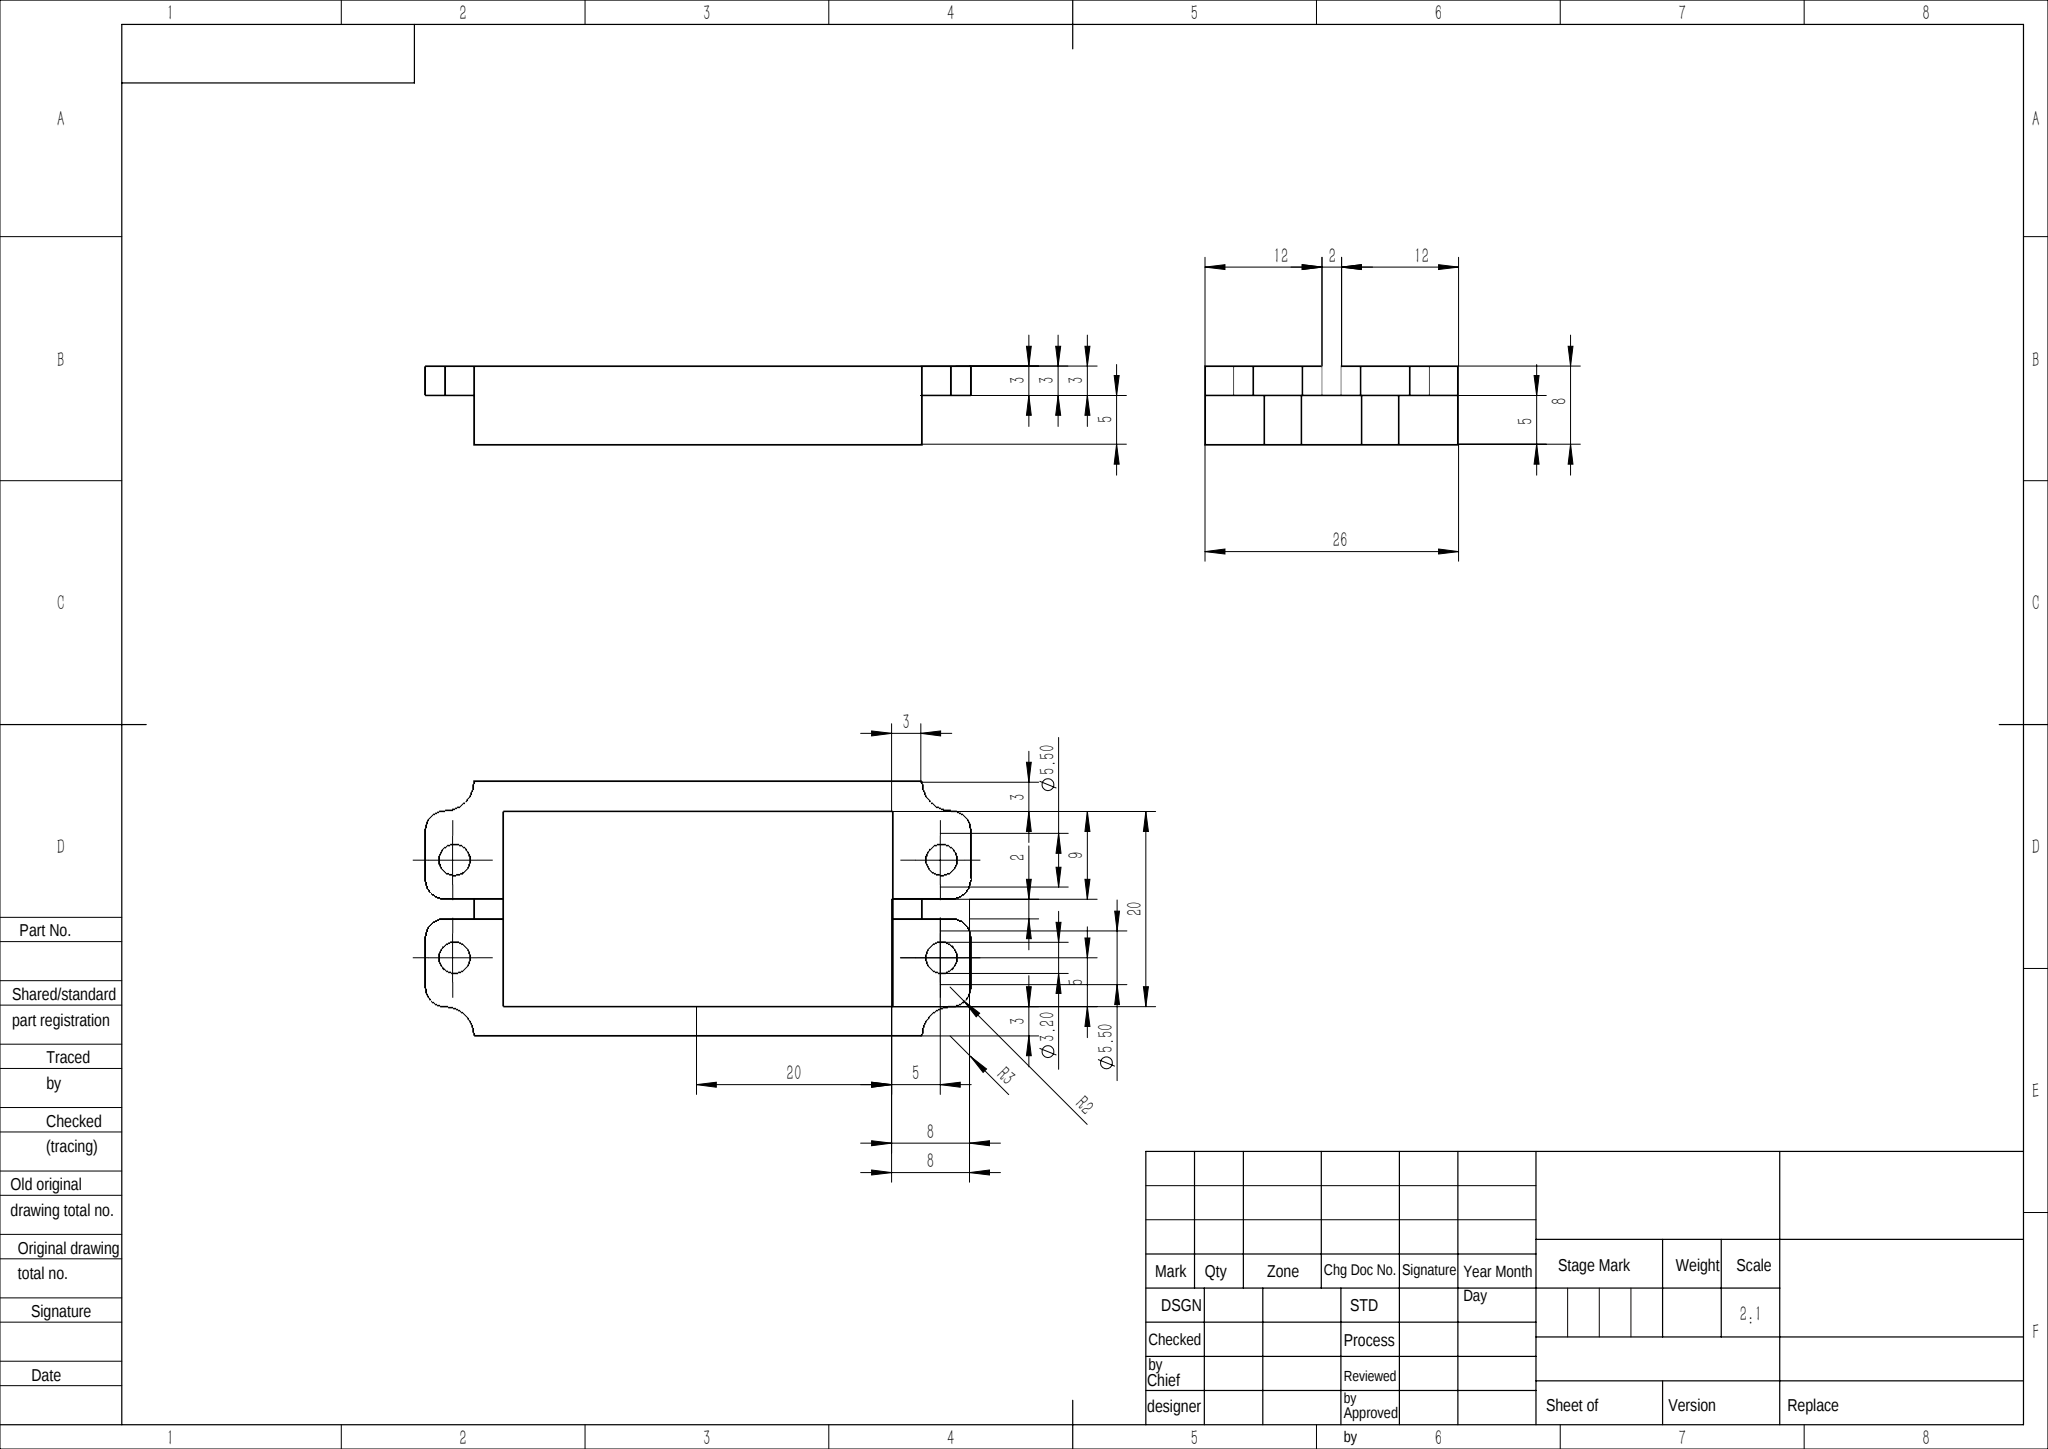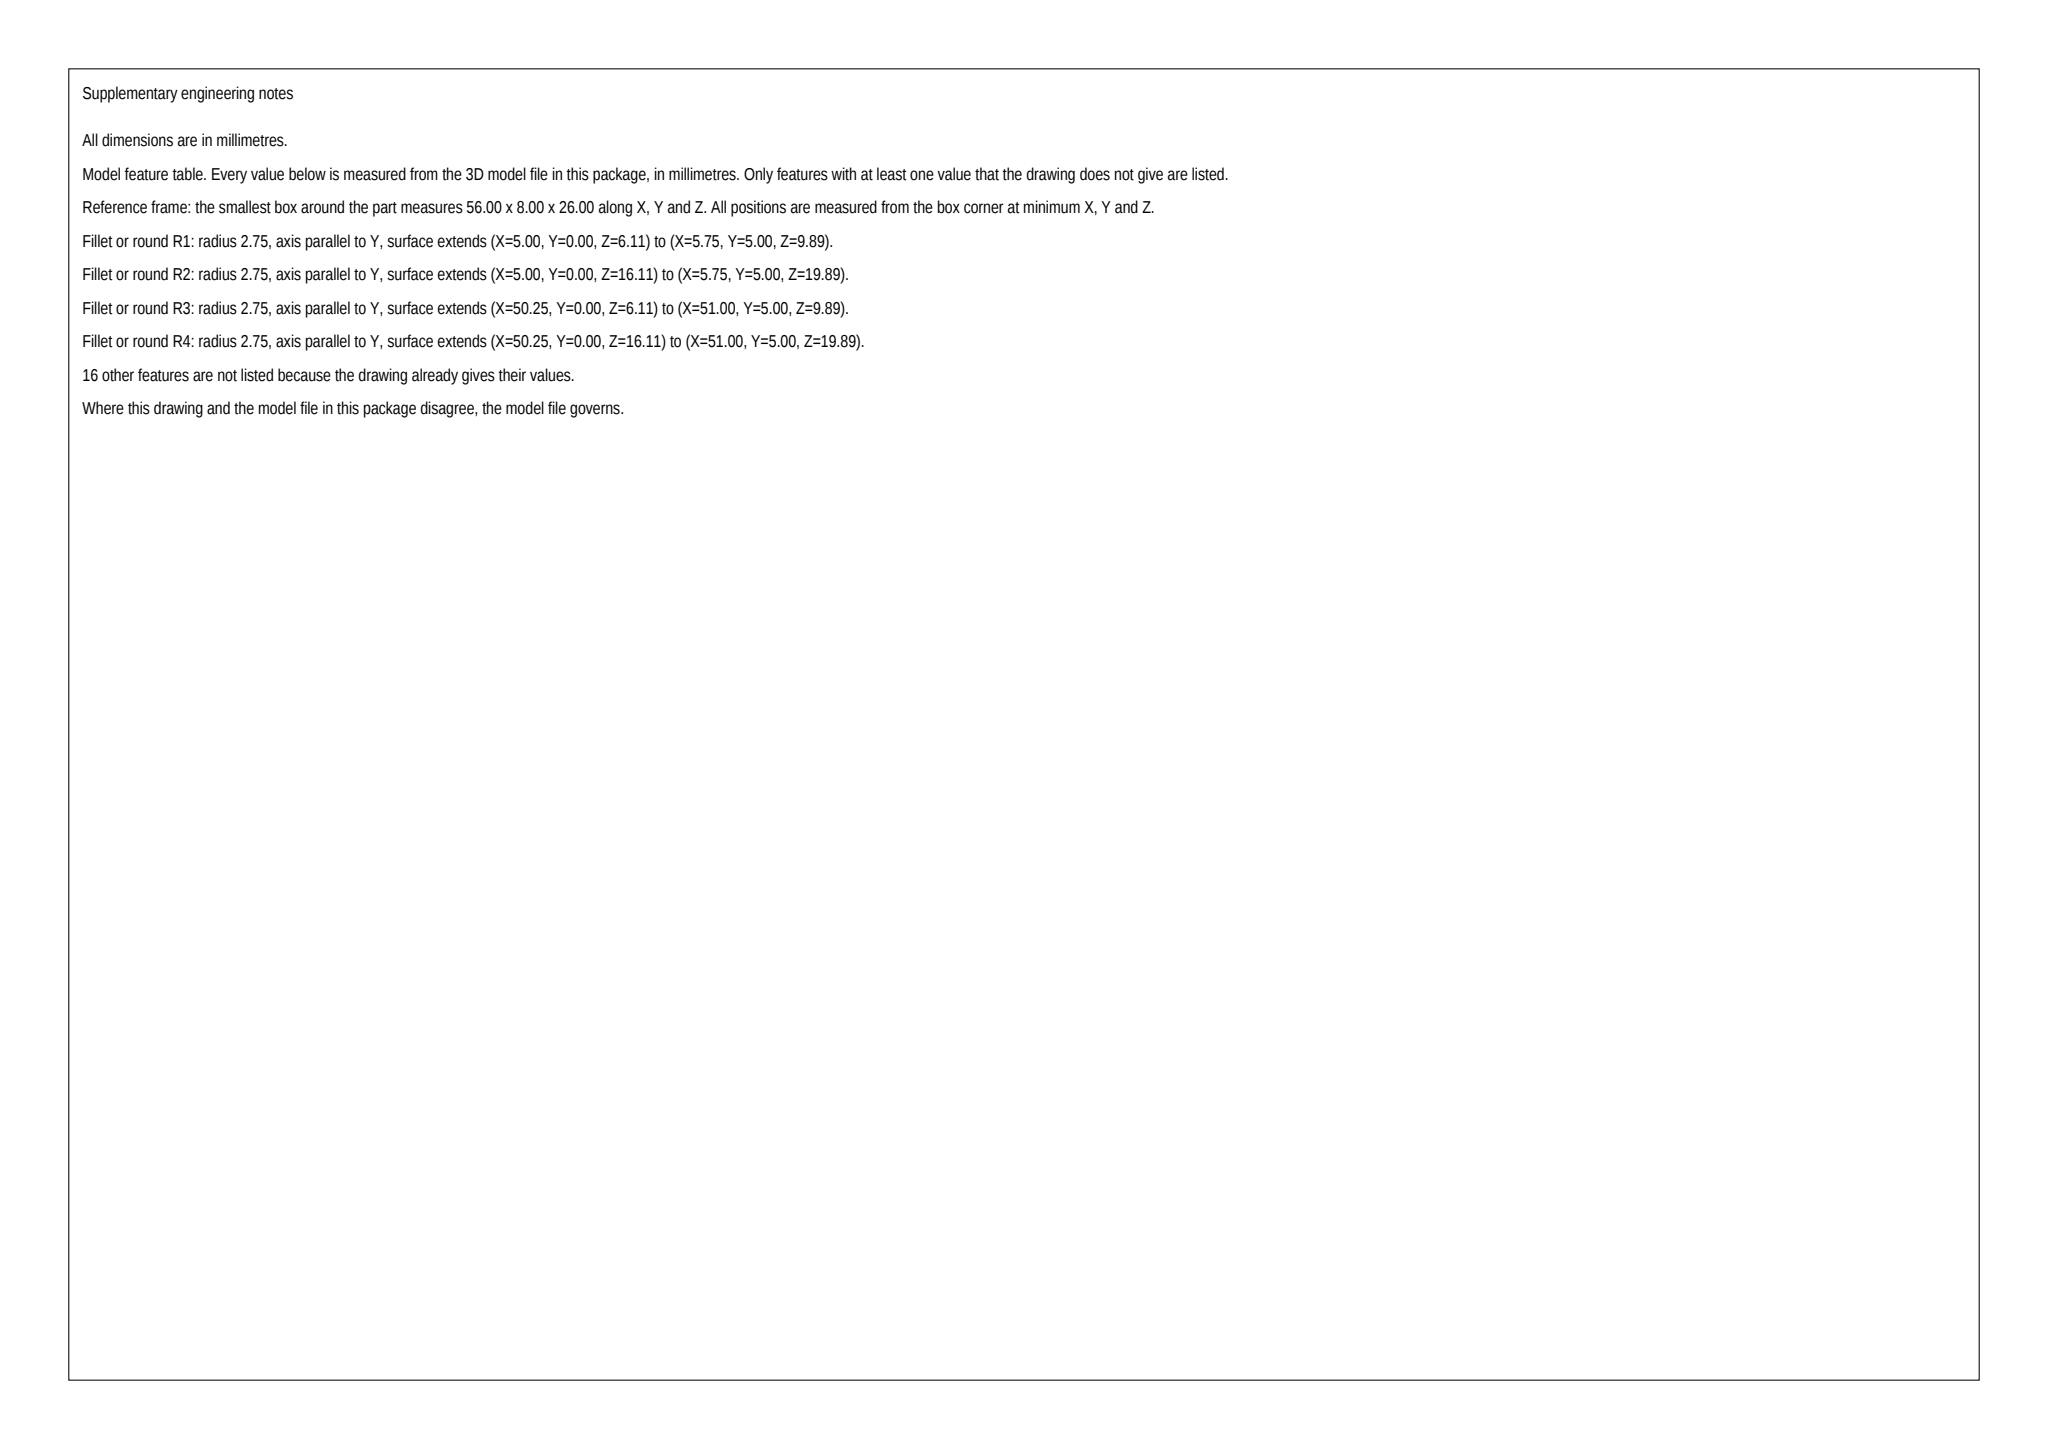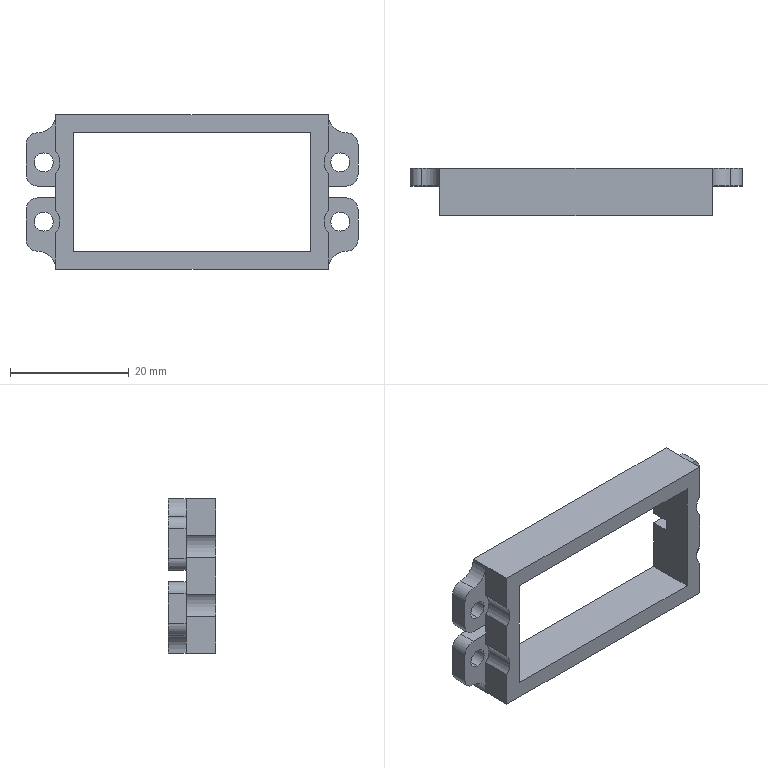Part | SolidWorks | mm | 1 solid | 53 faces | box 56 x 8 x 26 mm | volume 3539 mm3 | plane 29 | cylinder 24 | commonest cylinder face diameters 3.2 x8 4 x8 5.5 x4 6 x4